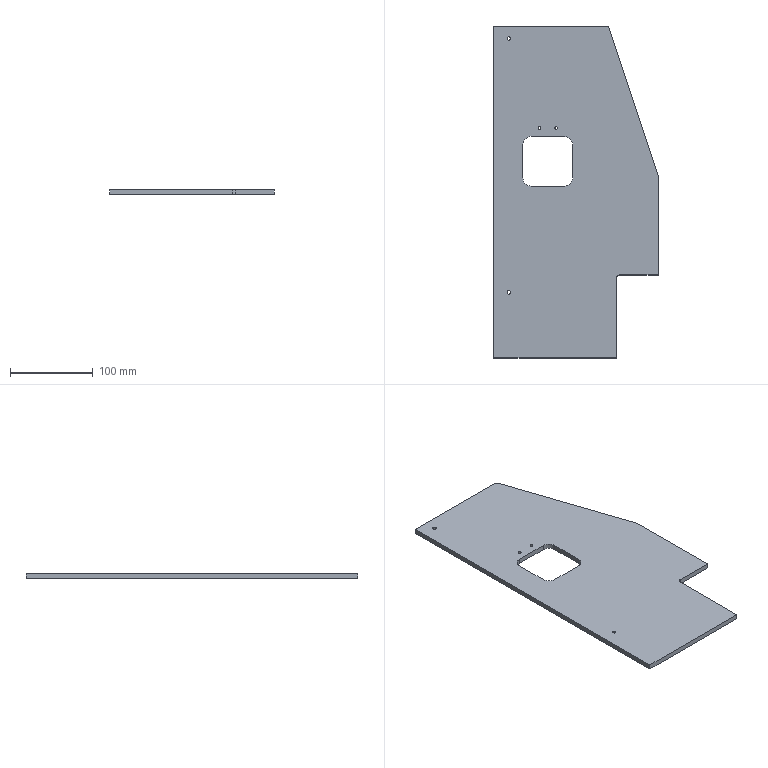Component | SolidWorks | THK-B1006RightFrontBaffle-1 | 1 solid | 28 faces | box 198 x 400 x 6 mm | volume 391453 mm3 | cylinder 15 | plane 13 | commonest cylinder face diameters 3.3 x4 4.2 x4 20 x4 8 x2 7 x1 | material Q235A
build123d program:
from build123d import *

# Parameters (mm, degrees)
BOSS_EXTRUDE1_DEPTH = 3
M5_TAPPED_HOLE1_D   = 4.2
FILLET1_R           = 4
M4_TAPPED_HOLE1_D   = 3.3


with BuildPart() as part:
    # Sketch1 → Boss-Extrude1 (new, symmetric)
    with BuildSketch(Plane(origin=(0, 0, 0), x_dir=(-1, 0, 0), z_dir=(0, 0, -1))):
        with BuildLine():
            Line((-99, 200), (39, 200))
            Line((39, 200), (99, 20))
            Line((99, 20), (99, -100))
            Line((99, -100), (52.5, -100))
            ThreePointArc((52.5, -100), (50.025, -101.025), (49, -103.5))
            Line((49, -103.5), (49, -200))
            Line((49, -200), (-99, -200))
            Line((-99, -200), (-99, 200))
        make_face()
        with BuildLine():
            Line((-14, 67), (-54, 67))
            ThreePointArc((-54, 67), (-61.071, 64.071), (-64, 57))
            Line((-64, 57), (-64, 17))
            ThreePointArc((-64, 17), (-61.071, 9.929), (-54, 7))
            Line((-54, 7), (-14, 7))
            ThreePointArc((-14, 7), (-6.929, 9.929), (-4, 17))
            Line((-4, 17), (-4, 57))
            ThreePointArc((-4, 57), (-6.929, 64.071), (-14, 67))
        make_face(mode=Mode.SUBTRACT)
    extrude(amount=BOSS_EXTRUDE1_DEPTH, both=True)

    # M5 Tapped Hole1 (through all)
    with Locations(Plane(origin=(0, 0, -3), x_dir=(-1, 0, 0), z_dir=(0, 0, -1))):
        with Locations((-81, 185), (-81, -121)):
            Hole(M5_TAPPED_HOLE1_D / 2)

    # Fillet1
    fillet1_edges = [part.edges().sort_by_distance(p)[0] for p in [
        (-39, 200, 0),
        (-99, 20, 0),
    ]]
    fillet(fillet1_edges, radius=FILLET1_R)

    # M4 Tapped Hole1 (through all)
    with Locations(Plane.XY.offset(3)):
        with Locations((24, 77), (44, 77)):
            Hole(M4_TAPPED_HOLE1_D / 2)


solid = part.part

# Placed as in the assembly
solid = solid.moved(Location((221, 0, -258), (-180, 0, 180)))
STEP:
#1=COLOUR_RGB('',0.7922,0.8196,0.9333);
#2=FILL_AREA_STYLE_COLOUR('',#1);
#3=FILL_AREA_STYLE('',(#2));
#4=SURFACE_STYLE_FILL_AREA(#3);
#5=SURFACE_SIDE_STYLE('',(#4));
#6=SURFACE_STYLE_USAGE(.BOTH.,#5);
#7=PRESENTATION_STYLE_ASSIGNMENT((#6));
#8=CARTESIAN_POINT('',(7.821,3.031,-10.039));
#9=VERTEX_POINT('',#8);
#10=CARTESIAN_POINT('',(7.691,3.031,-10.039));
#11=VERTEX_POINT('',#10);
#12=CARTESIAN_POINT('',(7.756,3.031,-10.039));
#13=DIRECTION('',(0.,-0.,-1.));
#14=DIRECTION('',(-1.,0.,0.));
#15=AXIS2_PLACEMENT_3D('',#12,#13,#14);
#16=CIRCLE('',#15,0.06496);
#17=EDGE_CURVE('',#9,#11,#16,.T.);
#18=ORIENTED_EDGE('',*,*,#17,.F.);
#19=CARTESIAN_POINT('',(7.821,3.031,-10.276));
#20=VERTEX_POINT('',#19);
#21=CARTESIAN_POINT('',(7.821,3.031,-10.276));
#22=DIRECTION('',(0.,-0.,-1.));
#23=VECTOR('',#22,39.37);
#24=LINE('',#21,#23);
#25=EDGE_CURVE('',#9,#20,#24,.T.);
#26=ORIENTED_EDGE('',*,*,#25,.T.);
#27=CARTESIAN_POINT('',(7.691,3.031,-10.276));
#28=VERTEX_POINT('',#27);
#29=CARTESIAN_POINT('',(7.756,3.031,-10.276));
#30=DIRECTION('',(0.,-0.,-1.));
#31=DIRECTION('',(-1.,0.,0.));
#32=AXIS2_PLACEMENT_3D('',#29,#30,#31);
#33=CIRCLE('',#32,0.06496);
#34=EDGE_CURVE('',#20,#28,#33,.T.);
#35=ORIENTED_EDGE('',*,*,#34,.T.);
#36=CARTESIAN_POINT('',(7.691,3.031,-10.276));
#37=DIRECTION('',(0.,-0.,-1.));
#38=VECTOR('',#37,39.37);
#39=LINE('',#36,#38);
#40=EDGE_CURVE('',#11,#28,#39,.T.);
#41=ORIENTED_EDGE('',*,*,#40,.F.);
#42=EDGE_LOOP('',(#18,#26,#35,#41));
#43=FACE_OUTER_BOUND('',#42,.T.);
#44=CARTESIAN_POINT('',(7.756,3.031,-10.276));
#45=DIRECTION('',(0.,-0.,-1.));
#46=DIRECTION('',(-1.,0.,0.));
#47=AXIS2_PLACEMENT_3D('',#44,#45,#46);
#48=CYLINDRICAL_SURFACE('',#47,0.06496);
#49=ADVANCED_FACE('',(#43),#48,.F.);
#50=CARTESIAN_POINT('',(7.033,3.031,-10.039));
#51=VERTEX_POINT('',#50);
#52=CARTESIAN_POINT('',(6.904,3.031,-10.039));
#53=VERTEX_POINT('',#52);
#54=CARTESIAN_POINT('',(6.969,3.031,-10.039));
#55=DIRECTION('',(0.,-0.,-1.));
#56=DIRECTION('',(-1.,0.,0.));
#57=AXIS2_PLACEMENT_3D('',#54,#55,#56);
#58=CIRCLE('',#57,0.06496);
#59=EDGE_CURVE('',#51,#53,#58,.T.);
#60=ORIENTED_EDGE('',*,*,#59,.F.);
#61=CARTESIAN_POINT('',(7.033,3.031,-10.276));
#62=VERTEX_POINT('',#61);
#63=CARTESIAN_POINT('',(7.033,3.031,-10.276));
#64=DIRECTION('',(0.,-0.,-1.));
#65=VECTOR('',#64,39.37);
#66=LINE('',#63,#65);
#67=EDGE_CURVE('',#51,#62,#66,.T.);
#68=ORIENTED_EDGE('',*,*,#67,.T.);
#69=CARTESIAN_POINT('',(6.904,3.031,-10.276));
#70=VERTEX_POINT('',#69);
#71=CARTESIAN_POINT('',(6.969,3.031,-10.276));
#72=DIRECTION('',(0.,-0.,-1.));
#73=DIRECTION('',(-1.,0.,0.));
#74=AXIS2_PLACEMENT_3D('',#71,#72,#73);
#75=CIRCLE('',#74,0.06496);
#76=EDGE_CURVE('',#62,#70,#75,.T.);
#77=ORIENTED_EDGE('',*,*,#76,.T.);
#78=CARTESIAN_POINT('',(6.904,3.031,-10.276));
#79=DIRECTION('',(0.,-0.,-1.));
#80=VECTOR('',#79,39.37);
#81=LINE('',#78,#80);
#82=EDGE_CURVE('',#53,#70,#81,.T.);
#83=ORIENTED_EDGE('',*,*,#82,.F.);
#84=EDGE_LOOP('',(#60,#68,#77,#83));
#85=FACE_OUTER_BOUND('',#84,.T.);
#86=CARTESIAN_POINT('',(6.969,3.031,-10.276));
#87=DIRECTION('',(0.,-0.,-1.));
#88=DIRECTION('',(-1.,0.,0.));
#89=AXIS2_PLACEMENT_3D('',#86,#87,#88);
#90=CYLINDRICAL_SURFACE('',#89,0.06496);
#91=ADVANCED_FACE('',(#85),#90,.F.);
#92=CARTESIAN_POINT('',(5.429,7.283,-10.276));
#93=VERTEX_POINT('',#92);
#94=CARTESIAN_POINT('',(5.594,7.283,-10.276));
#95=VERTEX_POINT('',#94);
#96=CARTESIAN_POINT('',(5.512,7.283,-10.276));
#97=DIRECTION('',(-0.,0.,1.));
#98=DIRECTION('',(1.,0.,0.));
#99=AXIS2_PLACEMENT_3D('',#96,#97,#98);
#100=CIRCLE('',#99,0.08268);
#101=EDGE_CURVE('',#93,#95,#100,.T.);
#102=ORIENTED_EDGE('',*,*,#101,.F.);
#103=CARTESIAN_POINT('',(5.429,7.283,-10.039));
#104=VERTEX_POINT('',#103);
#105=CARTESIAN_POINT('',(5.429,7.283,-10.039));
#106=DIRECTION('',(-0.,0.,1.));
#107=VECTOR('',#106,39.37);
#108=LINE('',#105,#107);
#109=EDGE_CURVE('',#93,#104,#108,.T.);
#110=ORIENTED_EDGE('',*,*,#109,.T.);
#111=CARTESIAN_POINT('',(5.594,7.283,-10.039));
#112=VERTEX_POINT('',#111);
#113=CARTESIAN_POINT('',(5.512,7.283,-10.039));
#114=DIRECTION('',(-0.,0.,1.));
#115=DIRECTION('',(1.,0.,0.));
#116=AXIS2_PLACEMENT_3D('',#113,#114,#115);
#117=CIRCLE('',#116,0.08268);
#118=EDGE_CURVE('',#104,#112,#117,.T.);
#119=ORIENTED_EDGE('',*,*,#118,.T.);
#120=CARTESIAN_POINT('',(5.594,7.283,-10.039));
#121=DIRECTION('',(-0.,0.,1.));
#122=VECTOR('',#121,39.37);
#123=LINE('',#120,#122);
#124=EDGE_CURVE('',#95,#112,#123,.T.);
#125=ORIENTED_EDGE('',*,*,#124,.F.);
#126=EDGE_LOOP('',(#102,#110,#119,#125));
#127=FACE_OUTER_BOUND('',#126,.T.);
#128=CARTESIAN_POINT('',(5.512,7.283,-10.039));
#129=DIRECTION('',(-0.,0.,1.));
#130=DIRECTION('',(1.,0.,0.));
#131=AXIS2_PLACEMENT_3D('',#128,#129,#130);
#132=CYLINDRICAL_SURFACE('',#131,0.08268);
#133=ADVANCED_FACE('',(#127),#132,.F.);
#134=CARTESIAN_POINT('',(5.429,-4.764,-10.276));
#135=VERTEX_POINT('',#134);
#136=CARTESIAN_POINT('',(5.594,-4.764,-10.276));
#137=VERTEX_POINT('',#136);
#138=CARTESIAN_POINT('',(5.512,-4.764,-10.276));
#139=DIRECTION('',(-0.,0.,1.));
#140=DIRECTION('',(1.,0.,0.));
#141=AXIS2_PLACEMENT_3D('',#138,#139,#140);
#142=CIRCLE('',#141,0.08268);
#143=EDGE_CURVE('',#135,#137,#142,.T.);
#144=ORIENTED_EDGE('',*,*,#143,.F.);
#145=CARTESIAN_POINT('',(5.429,-4.764,-10.039));
#146=VERTEX_POINT('',#145);
#147=CARTESIAN_POINT('',(5.429,-4.764,-10.039));
#148=DIRECTION('',(-0.,0.,1.));
#149=VECTOR('',#148,39.37);
#150=LINE('',#147,#149);
#151=EDGE_CURVE('',#135,#146,#150,.T.);
#152=ORIENTED_EDGE('',*,*,#151,.T.);
#153=CARTESIAN_POINT('',(5.594,-4.764,-10.039));
#154=VERTEX_POINT('',#153);
#155=CARTESIAN_POINT('',(5.512,-4.764,-10.039));
#156=DIRECTION('',(-0.,0.,1.));
#157=DIRECTION('',(1.,0.,0.));
#158=AXIS2_PLACEMENT_3D('',#155,#156,#157);
#159=CIRCLE('',#158,0.08268);
#160=EDGE_CURVE('',#146,#154,#159,.T.);
#161=ORIENTED_EDGE('',*,*,#160,.T.);
#162=CARTESIAN_POINT('',(5.594,-4.764,-10.039));
#163=DIRECTION('',(-0.,0.,1.));
#164=VECTOR('',#163,39.37);
#165=LINE('',#162,#164);
#166=EDGE_CURVE('',#137,#154,#165,.T.);
#167=ORIENTED_EDGE('',*,*,#166,.F.);
#168=EDGE_LOOP('',(#144,#152,#161,#167));
#169=FACE_OUTER_BOUND('',#168,.T.);
#170=CARTESIAN_POINT('',(5.512,-4.764,-10.039));
#171=DIRECTION('',(-0.,0.,1.));
#172=DIRECTION('',(1.,0.,0.));
#173=AXIS2_PLACEMENT_3D('',#170,#171,#172);
#174=CYLINDRICAL_SURFACE('',#173,0.08268);
#175=ADVANCED_FACE('',(#169),#174,.F.);
#176=CARTESIAN_POINT('',(7.756,3.031,-10.039));
#177=DIRECTION('',(0.,-0.,-1.));
#178=DIRECTION('',(-1.,0.,0.));
#179=AXIS2_PLACEMENT_3D('',#176,#177,#178);
#180=CIRCLE('',#179,0.06496);
#181=EDGE_CURVE('',#11,#9,#180,.T.);
#182=ORIENTED_EDGE('',*,*,#181,.T.);
#183=ORIENTED_EDGE('',*,*,#17,.T.);
#184=EDGE_LOOP('',(#182,#183));
#185=FACE_BOUND('',#184,.T.);
#186=CARTESIAN_POINT('',(6.969,3.031,-10.039));
#187=DIRECTION('',(0.,-0.,-1.));
#188=DIRECTION('',(-1.,0.,0.));
#189=AXIS2_PLACEMENT_3D('',#186,#187,#188);
#190=CIRCLE('',#189,0.06496);
#191=EDGE_CURVE('',#53,#51,#190,.T.);
#192=ORIENTED_EDGE('',*,*,#191,.T.);
#193=ORIENTED_EDGE('',*,*,#59,.T.);
#194=EDGE_LOOP('',(#192,#193));
#195=FACE_BOUND('',#194,.T.);
#196=CARTESIAN_POINT('',(5.512,7.283,-10.039));
#197=DIRECTION('',(-0.,0.,1.));
#198=DIRECTION('',(1.,0.,0.));
#199=AXIS2_PLACEMENT_3D('',#196,#197,#198);
#200=CIRCLE('',#199,0.08268);
#201=EDGE_CURVE('',#112,#104,#200,.T.);
#202=ORIENTED_EDGE('',*,*,#201,.F.);
#203=ORIENTED_EDGE('',*,*,#118,.F.);
#204=EDGE_LOOP('',(#202,#203));
#205=FACE_BOUND('',#204,.T.);
#206=CARTESIAN_POINT('',(5.512,-4.764,-10.039));
#207=DIRECTION('',(-0.,0.,1.));
#208=DIRECTION('',(1.,0.,0.));
#209=AXIS2_PLACEMENT_3D('',#206,#207,#208);
#210=CIRCLE('',#209,0.08268);
#211=EDGE_CURVE('',#154,#146,#210,.T.);
#212=ORIENTED_EDGE('',*,*,#211,.F.);
#213=ORIENTED_EDGE('',*,*,#160,.F.);
#214=EDGE_LOOP('',(#212,#213));
#215=FACE_BOUND('',#214,.T.);
#216=CARTESIAN_POINT('',(12.598,-3.937,-10.039));
#217=VERTEX_POINT('',#216);
#218=CARTESIAN_POINT('',(12.598,0.7618,-10.039));
#219=VERTEX_POINT('',#218);
#220=CARTESIAN_POINT('',(12.598,0.7874,-10.039));
#221=DIRECTION('',(-0.,1.,-0.));
#222=VECTOR('',#221,39.37);
#223=LINE('',#220,#222);
#224=EDGE_CURVE('',#217,#219,#223,.T.);
#225=ORIENTED_EDGE('',*,*,#224,.T.);
#226=CARTESIAN_POINT('',(12.59,0.8116,-10.039));
#227=VERTEX_POINT('',#226);
#228=CARTESIAN_POINT('',(12.441,0.7618,-10.039));
#229=DIRECTION('',(-0.,0.,1.));
#230=DIRECTION('',(-1.,0.,0.));
#231=AXIS2_PLACEMENT_3D('',#228,#229,#230);
#232=CIRCLE('',#231,0.1575);
#233=EDGE_CURVE('',#219,#227,#232,.T.);
#234=ORIENTED_EDGE('',*,*,#233,.T.);
#235=CARTESIAN_POINT('',(10.272,7.766,-10.039));
#236=VERTEX_POINT('',#235);
#237=CARTESIAN_POINT('',(10.236,7.874,-10.039));
#238=DIRECTION('',(-0.3162,0.9487,-0.));
#239=VECTOR('',#238,39.37);
#240=LINE('',#237,#239);
#241=EDGE_CURVE('',#227,#236,#240,.T.);
#242=ORIENTED_EDGE('',*,*,#241,.T.);
#243=CARTESIAN_POINT('',(10.123,7.874,-10.039));
#244=VERTEX_POINT('',#243);
#245=CARTESIAN_POINT('',(10.123,7.717,-10.039));
#246=DIRECTION('',(-0.,0.,1.));
#247=DIRECTION('',(-1.,0.,0.));
#248=AXIS2_PLACEMENT_3D('',#245,#246,#247);
#249=CIRCLE('',#248,0.1575);
#250=EDGE_CURVE('',#236,#244,#249,.T.);
#251=ORIENTED_EDGE('',*,*,#250,.T.);
#252=CARTESIAN_POINT('',(4.803,7.874,-10.039));
#253=VERTEX_POINT('',#252);
#254=CARTESIAN_POINT('',(4.803,7.874,-10.039));
#255=DIRECTION('',(-1.,0.,-0.));
#256=VECTOR('',#255,39.37);
#257=LINE('',#254,#256);
#258=EDGE_CURVE('',#244,#253,#257,.T.);
#259=ORIENTED_EDGE('',*,*,#258,.T.);
#260=CARTESIAN_POINT('',(4.803,-7.874,-10.039));
#261=VERTEX_POINT('',#260);
#262=CARTESIAN_POINT('',(4.803,-7.874,-10.039));
#263=DIRECTION('',(0.,-1.,0.));
#264=VECTOR('',#263,39.37);
#265=LINE('',#262,#264);
#266=EDGE_CURVE('',#253,#261,#265,.T.);
#267=ORIENTED_EDGE('',*,*,#266,.T.);
#268=CARTESIAN_POINT('',(10.63,-7.874,-10.039));
#269=VERTEX_POINT('',#268);
#270=CARTESIAN_POINT('',(10.63,-7.874,-10.039));
#271=DIRECTION('',(1.,0.,0.));
#272=VECTOR('',#271,39.37);
#273=LINE('',#270,#272);
#274=EDGE_CURVE('',#261,#269,#273,.T.);
#275=ORIENTED_EDGE('',*,*,#274,.T.);
#276=CARTESIAN_POINT('',(10.63,-4.075,-10.039));
#277=VERTEX_POINT('',#276);
#278=CARTESIAN_POINT('',(10.63,-7.874,-10.039));
#279=DIRECTION('',(-0.,1.,-0.));
#280=VECTOR('',#279,39.37);
#281=LINE('',#278,#280);
#282=EDGE_CURVE('',#269,#277,#281,.T.);
#283=ORIENTED_EDGE('',*,*,#282,.T.);
#284=CARTESIAN_POINT('',(10.768,-3.937,-10.039));
#285=VERTEX_POINT('',#284);
#286=CARTESIAN_POINT('',(10.768,-4.075,-10.039));
#287=DIRECTION('',(0.,-0.,-1.));
#288=DIRECTION('',(-1.,0.,0.));
#289=AXIS2_PLACEMENT_3D('',#286,#287,#288);
#290=CIRCLE('',#289,0.1378);
#291=EDGE_CURVE('',#277,#285,#290,.T.);
#292=ORIENTED_EDGE('',*,*,#291,.T.);
#293=CARTESIAN_POINT('',(10.768,-3.937,-10.039));
#294=DIRECTION('',(1.,0.,0.));
#295=VECTOR('',#294,39.37);
#296=LINE('',#293,#295);
#297=EDGE_CURVE('',#285,#217,#296,.T.);
#298=ORIENTED_EDGE('',*,*,#297,.T.);
#299=EDGE_LOOP('',(#225,#234,#242,#251,#259,#267,#275,#283,#292,#298));
#300=FACE_OUTER_BOUND('',#299,.T.);
#301=CARTESIAN_POINT('',(6.575,2.638,-10.039));
#302=VERTEX_POINT('',#301);
#303=CARTESIAN_POINT('',(6.181,2.244,-10.039));
#304=VERTEX_POINT('',#303);
#305=CARTESIAN_POINT('',(6.575,2.244,-10.039));
#306=DIRECTION('',(-0.,0.,1.));
#307=DIRECTION('',(1.,0.,0.));
#308=AXIS2_PLACEMENT_3D('',#305,#306,#307);
#309=CIRCLE('',#308,0.3937);
#310=EDGE_CURVE('',#302,#304,#309,.T.);
#311=ORIENTED_EDGE('',*,*,#310,.F.);
#312=CARTESIAN_POINT('',(8.15,2.638,-10.039));
#313=VERTEX_POINT('',#312);
#314=CARTESIAN_POINT('',(8.15,2.638,-10.039));
#315=DIRECTION('',(-1.,-0.,-0.));
#316=VECTOR('',#315,39.37);
#317=LINE('',#314,#316);
#318=EDGE_CURVE('',#313,#302,#317,.T.);
#319=ORIENTED_EDGE('',*,*,#318,.F.);
#320=CARTESIAN_POINT('',(8.543,2.244,-10.039));
#321=VERTEX_POINT('',#320);
#322=CARTESIAN_POINT('',(8.15,2.244,-10.039));
#323=DIRECTION('',(-0.,0.,1.));
#324=DIRECTION('',(1.,0.,0.));
#325=AXIS2_PLACEMENT_3D('',#322,#323,#324);
#326=CIRCLE('',#325,0.3937);
#327=EDGE_CURVE('',#321,#313,#326,.T.);
#328=ORIENTED_EDGE('',*,*,#327,.F.);
#329=CARTESIAN_POINT('',(8.543,0.6693,-10.039));
#330=VERTEX_POINT('',#329);
#331=CARTESIAN_POINT('',(8.543,2.244,-10.039));
#332=DIRECTION('',(-0.,1.,-0.));
#333=VECTOR('',#332,39.37);
#334=LINE('',#331,#333);
#335=EDGE_CURVE('',#330,#321,#334,.T.);
#336=ORIENTED_EDGE('',*,*,#335,.F.);
#337=CARTESIAN_POINT('',(8.15,0.2756,-10.039));
#338=VERTEX_POINT('',#337);
#339=CARTESIAN_POINT('',(8.15,0.6693,-10.039));
#340=DIRECTION('',(-0.,0.,1.));
#341=DIRECTION('',(-1.,0.,0.));
#342=AXIS2_PLACEMENT_3D('',#339,#340,#341);
#343=CIRCLE('',#342,0.3937);
#344=EDGE_CURVE('',#338,#330,#343,.T.);
#345=ORIENTED_EDGE('',*,*,#344,.F.);
#346=CARTESIAN_POINT('',(6.575,0.2756,-10.039));
#347=VERTEX_POINT('',#346);
#348=CARTESIAN_POINT('',(8.15,0.2756,-10.039));
#349=DIRECTION('',(1.,0.,0.));
#350=VECTOR('',#349,39.37);
#351=LINE('',#348,#350);
#352=EDGE_CURVE('',#347,#338,#351,.T.);
#353=ORIENTED_EDGE('',*,*,#352,.F.);
#354=CARTESIAN_POINT('',(6.181,0.6693,-10.039));
#355=VERTEX_POINT('',#354);
#356=CARTESIAN_POINT('',(6.575,0.6693,-10.039));
#357=DIRECTION('',(-0.,0.,1.));
#358=DIRECTION('',(1.,0.,0.));
#359=AXIS2_PLACEMENT_3D('',#356,#357,#358);
#360=CIRCLE('',#359,0.3937);
#361=EDGE_CURVE('',#355,#347,#360,.T.);
#362=ORIENTED_EDGE('',*,*,#361,.F.);
#363=CARTESIAN_POINT('',(6.181,2.244,-10.039));
#364=DIRECTION('',(0.,-1.,0.));
#365=VECTOR('',#364,39.37);
#366=LINE('',#363,#365);
#367=EDGE_CURVE('',#304,#355,#366,.T.);
#368=ORIENTED_EDGE('',*,*,#367,.F.);
#369=EDGE_LOOP('',(#311,#319,#328,#336,#345,#353,#362,#368));
#370=FACE_BOUND('',#369,.T.);
#371=CARTESIAN_POINT('',(10.768,-4.075,-10.039));
#372=DIRECTION('',(0.,-0.,-1.));
#373=DIRECTION('',(-1.,-0.,-0.));
#374=AXIS2_PLACEMENT_3D('',#371,#372,#373);
#375=PLANE('',#374);
#376=ADVANCED_FACE('',(#185,#195,#205,#215,#300,#370),#375,.F.);
#377=CARTESIAN_POINT('',(7.756,3.031,-10.276));
#378=DIRECTION('',(0.,-0.,-1.));
#379=DIRECTION('',(-1.,0.,0.));
#380=AXIS2_PLACEMENT_3D('',#377,#378,#379);
#381=CIRCLE('',#380,0.06496);
#382=EDGE_CURVE('',#28,#20,#381,.T.);
#383=ORIENTED_EDGE('',*,*,#382,.F.);
#384=ORIENTED_EDGE('',*,*,#34,.F.);
#385=EDGE_LOOP('',(#383,#384));
#386=FACE_BOUND('',#385,.T.);
#387=CARTESIAN_POINT('',(6.969,3.031,-10.276));
#388=DIRECTION('',(0.,-0.,-1.));
#389=DIRECTION('',(-1.,0.,0.));
#390=AXIS2_PLACEMENT_3D('',#387,#388,#389);
#391=CIRCLE('',#390,0.06496);
#392=EDGE_CURVE('',#70,#62,#391,.T.);
#393=ORIENTED_EDGE('',*,*,#392,.F.);
#394=ORIENTED_EDGE('',*,*,#76,.F.);
#395=EDGE_LOOP('',(#393,#394));
#396=FACE_BOUND('',#395,.T.);
#397=CARTESIAN_POINT('',(5.512,7.283,-10.276));
#398=DIRECTION('',(-0.,0.,1.));
#399=DIRECTION('',(1.,0.,0.));
#400=AXIS2_PLACEMENT_3D('',#397,#398,#399);
#401=CIRCLE('',#400,0.08268);
#402=EDGE_CURVE('',#95,#93,#401,.T.);
#403=ORIENTED_EDGE('',*,*,#402,.T.);
#404=ORIENTED_EDGE('',*,*,#101,.T.);
#405=EDGE_LOOP('',(#403,#404));
#406=FACE_BOUND('',#405,.T.);
#407=CARTESIAN_POINT('',(5.512,-4.764,-10.276));
#408=DIRECTION('',(-0.,0.,1.));
#409=DIRECTION('',(1.,0.,0.));
#410=AXIS2_PLACEMENT_3D('',#407,#408,#409);
#411=CIRCLE('',#410,0.08268);
#412=EDGE_CURVE('',#137,#135,#411,.T.);
#413=ORIENTED_EDGE('',*,*,#412,.T.);
#414=ORIENTED_EDGE('',*,*,#143,.T.);
#415=EDGE_LOOP('',(#413,#414));
#416=FACE_BOUND('',#415,.T.);
#417=CARTESIAN_POINT('',(12.59,0.8116,-10.276));
#418=VERTEX_POINT('',#417);
#419=CARTESIAN_POINT('',(10.272,7.766,-10.276));
#420=VERTEX_POINT('',#419);
#421=CARTESIAN_POINT('',(10.236,7.874,-10.276));
#422=DIRECTION('',(-0.3162,0.9487,-0.));
#423=VECTOR('',#422,39.37);
#424=LINE('',#421,#423);
#425=EDGE_CURVE('',#418,#420,#424,.T.);
#426=ORIENTED_EDGE('',*,*,#425,.F.);
#427=CARTESIAN_POINT('',(12.598,0.7618,-10.276));
#428=VERTEX_POINT('',#427);
#429=CARTESIAN_POINT('',(12.441,0.7618,-10.276));
#430=DIRECTION('',(0.,-0.,-1.));
#431=DIRECTION('',(-1.,0.,0.));
#432=AXIS2_PLACEMENT_3D('',#429,#430,#431);
#433=CIRCLE('',#432,0.1575);
#434=EDGE_CURVE('',#418,#428,#433,.T.);
#435=ORIENTED_EDGE('',*,*,#434,.T.);
#436=CARTESIAN_POINT('',(12.598,-3.937,-10.276));
#437=VERTEX_POINT('',#436);
#438=CARTESIAN_POINT('',(12.598,0.7874,-10.276));
#439=DIRECTION('',(-0.,1.,-0.));
#440=VECTOR('',#439,39.37);
#441=LINE('',#438,#440);
#442=EDGE_CURVE('',#437,#428,#441,.T.);
#443=ORIENTED_EDGE('',*,*,#442,.F.);
#444=CARTESIAN_POINT('',(10.768,-3.937,-10.276));
#445=VERTEX_POINT('',#444);
#446=CARTESIAN_POINT('',(10.768,-3.937,-10.276));
#447=DIRECTION('',(1.,0.,0.));
#448=VECTOR('',#447,39.37);
#449=LINE('',#446,#448);
#450=EDGE_CURVE('',#445,#437,#449,.T.);
#451=ORIENTED_EDGE('',*,*,#450,.F.);
#452=CARTESIAN_POINT('',(10.63,-4.075,-10.276));
#453=VERTEX_POINT('',#452);
#454=CARTESIAN_POINT('',(10.768,-4.075,-10.276));
#455=DIRECTION('',(0.,-0.,-1.));
#456=DIRECTION('',(-1.,0.,0.));
#457=AXIS2_PLACEMENT_3D('',#454,#455,#456);
#458=CIRCLE('',#457,0.1378);
#459=EDGE_CURVE('',#453,#445,#458,.T.);
#460=ORIENTED_EDGE('',*,*,#459,.F.);
#461=CARTESIAN_POINT('',(10.63,-7.874,-10.276));
#462=VERTEX_POINT('',#461);
#463=CARTESIAN_POINT('',(10.63,-7.874,-10.276));
#464=DIRECTION('',(-0.,1.,-0.));
#465=VECTOR('',#464,39.37);
#466=LINE('',#463,#465);
#467=EDGE_CURVE('',#462,#453,#466,.T.);
#468=ORIENTED_EDGE('',*,*,#467,.F.);
#469=CARTESIAN_POINT('',(4.803,-7.874,-10.276));
#470=VERTEX_POINT('',#469);
#471=CARTESIAN_POINT('',(10.63,-7.874,-10.276));
#472=DIRECTION('',(1.,0.,0.));
#473=VECTOR('',#472,39.37);
#474=LINE('',#471,#473);
#475=EDGE_CURVE('',#470,#462,#474,.T.);
#476=ORIENTED_EDGE('',*,*,#475,.F.);
#477=CARTESIAN_POINT('',(4.803,7.874,-10.276));
#478=VERTEX_POINT('',#477);
#479=CARTESIAN_POINT('',(4.803,-7.874,-10.276));
#480=DIRECTION('',(0.,-1.,0.));
#481=VECTOR('',#480,39.37);
#482=LINE('',#479,#481);
#483=EDGE_CURVE('',#478,#470,#482,.T.);
#484=ORIENTED_EDGE('',*,*,#483,.F.);
#485=CARTESIAN_POINT('',(10.123,7.874,-10.276));
#486=VERTEX_POINT('',#485);
#487=CARTESIAN_POINT('',(4.803,7.874,-10.276));
#488=DIRECTION('',(-1.,0.,-0.));
#489=VECTOR('',#488,39.37);
#490=LINE('',#487,#489);
#491=EDGE_CURVE('',#486,#478,#490,.T.);
#492=ORIENTED_EDGE('',*,*,#491,.F.);
#493=CARTESIAN_POINT('',(10.123,7.717,-10.276));
#494=DIRECTION('',(0.,-0.,-1.));
#495=DIRECTION('',(-1.,0.,0.));
#496=AXIS2_PLACEMENT_3D('',#493,#494,#495);
#497=CIRCLE('',#496,0.1575);
#498=EDGE_CURVE('',#486,#420,#497,.T.);
#499=ORIENTED_EDGE('',*,*,#498,.T.);
#500=EDGE_LOOP('',(#426,#435,#443,#451,#460,#468,#476,#484,#492,#499));
#501=FACE_OUTER_BOUND('',#500,.T.);
#502=CARTESIAN_POINT('',(8.15,2.638,-10.276));
#503=VERTEX_POINT('',#502);
#504=CARTESIAN_POINT('',(6.575,2.638,-10.276));
#505=VERTEX_POINT('',#504);
#506=CARTESIAN_POINT('',(8.15,2.638,-10.276));
#507=DIRECTION('',(-1.,-0.,-0.));
#508=VECTOR('',#507,39.37);
#509=LINE('',#506,#508);
#510=EDGE_CURVE('',#503,#505,#509,.T.);
#511=ORIENTED_EDGE('',*,*,#510,.T.);
#512=CARTESIAN_POINT('',(6.181,2.244,-10.276));
#513=VERTEX_POINT('',#512);
#514=CARTESIAN_POINT('',(6.575,2.244,-10.276));
#515=DIRECTION('',(-0.,0.,1.));
#516=DIRECTION('',(1.,0.,0.));
#517=AXIS2_PLACEMENT_3D('',#514,#515,#516);
#518=CIRCLE('',#517,0.3937);
#519=EDGE_CURVE('',#505,#513,#518,.T.);
#520=ORIENTED_EDGE('',*,*,#519,.T.);
#521=CARTESIAN_POINT('',(6.181,0.6693,-10.276));
#522=VERTEX_POINT('',#521);
#523=CARTESIAN_POINT('',(6.181,2.244,-10.276));
#524=DIRECTION('',(0.,-1.,0.));
#525=VECTOR('',#524,39.37);
#526=LINE('',#523,#525);
#527=EDGE_CURVE('',#513,#522,#526,.T.);
#528=ORIENTED_EDGE('',*,*,#527,.T.);
#529=CARTESIAN_POINT('',(6.575,0.2756,-10.276));
#530=VERTEX_POINT('',#529);
#531=CARTESIAN_POINT('',(6.575,0.6693,-10.276));
#532=DIRECTION('',(-0.,0.,1.));
#533=DIRECTION('',(1.,0.,0.));
#534=AXIS2_PLACEMENT_3D('',#531,#532,#533);
#535=CIRCLE('',#534,0.3937);
#536=EDGE_CURVE('',#522,#530,#535,.T.);
#537=ORIENTED_EDGE('',*,*,#536,.T.);
#538=CARTESIAN_POINT('',(8.15,0.2756,-10.276));
#539=VERTEX_POINT('',#538);
#540=CARTESIAN_POINT('',(8.15,0.2756,-10.276));
#541=DIRECTION('',(1.,0.,0.));
#542=VECTOR('',#541,39.37);
#543=LINE('',#540,#542);
#544=EDGE_CURVE('',#530,#539,#543,.T.);
#545=ORIENTED_EDGE('',*,*,#544,.T.);
#546=CARTESIAN_POINT('',(8.543,0.6693,-10.276));
#547=VERTEX_POINT('',#546);
#548=CARTESIAN_POINT('',(8.15,0.6693,-10.276));
#549=DIRECTION('',(-0.,0.,1.));
#550=DIRECTION('',(-1.,0.,0.));
#551=AXIS2_PLACEMENT_3D('',#548,#549,#550);
#552=CIRCLE('',#551,0.3937);
#553=EDGE_CURVE('',#539,#547,#552,.T.);
#554=ORIENTED_EDGE('',*,*,#553,.T.);
#555=CARTESIAN_POINT('',(8.543,2.244,-10.276));
#556=VERTEX_POINT('',#555);
#557=CARTESIAN_POINT('',(8.543,2.244,-10.276));
#558=DIRECTION('',(-0.,1.,-0.));
#559=VECTOR('',#558,39.37);
#560=LINE('',#557,#559);
#561=EDGE_CURVE('',#547,#556,#560,.T.);
#562=ORIENTED_EDGE('',*,*,#561,.T.);
#563=CARTESIAN_POINT('',(8.15,2.244,-10.276));
#564=DIRECTION('',(-0.,0.,1.));
#565=DIRECTION('',(1.,0.,0.));
#566=AXIS2_PLACEMENT_3D('',#563,#564,#565);
#567=CIRCLE('',#566,0.3937);
#568=EDGE_CURVE('',#556,#503,#567,.T.);
#569=ORIENTED_EDGE('',*,*,#568,.T.);
#570=EDGE_LOOP('',(#511,#520,#528,#537,#545,#554,#562,#569));
#571=FACE_BOUND('',#570,.T.);
#572=CARTESIAN_POINT('',(10.768,-4.075,-10.276));
#573=DIRECTION('',(0.,-0.,-1.));
#574=DIRECTION('',(-1.,-0.,-0.));
#575=AXIS2_PLACEMENT_3D('',#572,#573,#574);
#576=PLANE('',#575);
#577=ADVANCED_FACE('',(#386,#396,#406,#416,#501,#571),#576,.T.);
#578=ORIENTED_EDGE('',*,*,#442,.T.);
#579=CARTESIAN_POINT('',(12.598,0.7618,-10.039));
#580=DIRECTION('',(-0.,0.,1.));
#581=VECTOR('',#580,39.37);
#582=LINE('',#579,#581);
#583=EDGE_CURVE('',#428,#219,#582,.T.);
#584=ORIENTED_EDGE('',*,*,#583,.T.);
#585=ORIENTED_EDGE('',*,*,#224,.F.);
#586=CARTESIAN_POINT('',(12.598,-3.937,-10.039));
#587=DIRECTION('',(0.,-0.,-1.));
#588=VECTOR('',#587,39.37);
#589=LINE('',#586,#588);
#590=EDGE_CURVE('',#217,#437,#589,.T.);
#591=ORIENTED_EDGE('',*,*,#590,.T.);
#592=EDGE_LOOP('',(#578,#584,#585,#591));
#593=FACE_OUTER_BOUND('',#592,.T.);
#594=CARTESIAN_POINT('',(12.598,0.7874,-10.039));
#595=DIRECTION('',(-1.,-0.,-0.));
#596=DIRECTION('',(-0.,1.,-0.));
#597=AXIS2_PLACEMENT_3D('',#594,#595,#596);
#598=PLANE('',#597);
#599=ADVANCED_FACE('',(#593),#598,.F.);
#600=ORIENTED_EDGE('',*,*,#241,.F.);
#601=CARTESIAN_POINT('',(12.59,0.8116,-10.039));
#602=DIRECTION('',(0.,-0.,-1.));
#603=VECTOR('',#602,39.37);
#604=LINE('',#601,#603);
#605=EDGE_CURVE('',#227,#418,#604,.T.);
#606=ORIENTED_EDGE('',*,*,#605,.T.);
#607=ORIENTED_EDGE('',*,*,#425,.T.);
#608=CARTESIAN_POINT('',(10.272,7.766,-10.039));
#609=DIRECTION('',(-0.,0.,1.));
#610=VECTOR('',#609,39.37);
#611=LINE('',#608,#610);
#612=EDGE_CURVE('',#420,#236,#611,.T.);
#613=ORIENTED_EDGE('',*,*,#612,.T.);
#614=EDGE_LOOP('',(#600,#606,#607,#613));
#615=FACE_OUTER_BOUND('',#614,.T.);
#616=CARTESIAN_POINT('',(10.236,7.874,-10.039));
#617=DIRECTION('',(-0.9487,-0.3162,-0.));
#618=DIRECTION('',(-0.3162,0.9487,-0.));
#619=AXIS2_PLACEMENT_3D('',#616,#617,#618);
#620=PLANE('',#619);
#621=ADVANCED_FACE('',(#615),#620,.F.);
#622=ORIENTED_EDGE('',*,*,#258,.F.);
#623=CARTESIAN_POINT('',(10.123,7.874,-10.039));
#624=DIRECTION('',(0.,-0.,-1.));
#625=VECTOR('',#624,39.37);
#626=LINE('',#623,#625);
#627=EDGE_CURVE('',#244,#486,#626,.T.);
#628=ORIENTED_EDGE('',*,*,#627,.T.);
#629=ORIENTED_EDGE('',*,*,#491,.T.);
#630=CARTESIAN_POINT('',(4.803,7.874,-10.039));
#631=DIRECTION('',(0.,-0.,-1.));
#632=VECTOR('',#631,39.37);
#633=LINE('',#630,#632);
#634=EDGE_CURVE('',#253,#478,#633,.T.);
#635=ORIENTED_EDGE('',*,*,#634,.F.);
#636=EDGE_LOOP('',(#622,#628,#629,#635));
#637=FACE_OUTER_BOUND('',#636,.T.);
#638=CARTESIAN_POINT('',(4.803,7.874,-10.039));
#639=DIRECTION('',(-0.,-1.,0.));
#640=DIRECTION('',(-1.,0.,-0.));
#641=AXIS2_PLACEMENT_3D('',#638,#639,#640);
#642=PLANE('',#641);
#643=ADVANCED_FACE('',(#637),#642,.F.);
#644=ORIENTED_EDGE('',*,*,#483,.T.);
#645=CARTESIAN_POINT('',(4.803,-7.874,-10.039));
#646=DIRECTION('',(0.,-0.,-1.));
#647=VECTOR('',#646,39.37);
#648=LINE('',#645,#647);
#649=EDGE_CURVE('',#261,#470,#648,.T.);
#650=ORIENTED_EDGE('',*,*,#649,.F.);
#651=ORIENTED_EDGE('',*,*,#266,.F.);
#652=ORIENTED_EDGE('',*,*,#634,.T.);
#653=EDGE_LOOP('',(#644,#650,#651,#652));
#654=FACE_OUTER_BOUND('',#653,.T.);
#655=CARTESIAN_POINT('',(4.803,-7.874,-10.039));
#656=DIRECTION('',(1.,0.,0.));
#657=DIRECTION('',(0.,-0.,-1.));
#658=AXIS2_PLACEMENT_3D('',#655,#656,#657);
#659=PLANE('',#658);
#660=ADVANCED_FACE('',(#654),#659,.F.);
#661=ORIENTED_EDGE('',*,*,#475,.T.);
#662=CARTESIAN_POINT('',(10.63,-7.874,-10.039));
#663=DIRECTION('',(0.,-0.,-1.));
#664=VECTOR('',#663,39.37);
#665=LINE('',#662,#664);
#666=EDGE_CURVE('',#269,#462,#665,.T.);
#667=ORIENTED_EDGE('',*,*,#666,.F.);
#668=ORIENTED_EDGE('',*,*,#274,.F.);
#669=ORIENTED_EDGE('',*,*,#649,.T.);
#670=EDGE_LOOP('',(#661,#667,#668,#669));
#671=FACE_OUTER_BOUND('',#670,.T.);
#672=CARTESIAN_POINT('',(10.63,-7.874,-10.039));
#673=DIRECTION('',(-0.,1.,-0.));
#674=DIRECTION('',(1.,0.,0.));
#675=AXIS2_PLACEMENT_3D('',#672,#673,#674);
#676=PLANE('',#675);
#677=ADVANCED_FACE('',(#671),#676,.F.);
#678=ORIENTED_EDGE('',*,*,#467,.T.);
#679=CARTESIAN_POINT('',(10.63,-4.075,-10.039));
#680=DIRECTION('',(0.,-0.,-1.));
#681=VECTOR('',#680,39.37);
#682=LINE('',#679,#681);
#683=EDGE_CURVE('',#277,#453,#682,.T.);
#684=ORIENTED_EDGE('',*,*,#683,.F.);
#685=ORIENTED_EDGE('',*,*,#282,.F.);
#686=ORIENTED_EDGE('',*,*,#666,.T.);
#687=EDGE_LOOP('',(#678,#684,#685,#686));
#688=FACE_OUTER_BOUND('',#687,.T.);
#689=CARTESIAN_POINT('',(10.63,-7.874,-10.039));
#690=DIRECTION('',(-1.,-0.,-0.));
#691=DIRECTION('',(-0.,0.,1.));
#692=AXIS2_PLACEMENT_3D('',#689,#690,#691);
#693=PLANE('',#692);
#694=ADVANCED_FACE('',(#688),#693,.F.);
#695=ORIENTED_EDGE('',*,*,#459,.T.);
#696=CARTESIAN_POINT('',(10.768,-3.937,-10.039));
#697=DIRECTION('',(0.,-0.,-1.));
#698=VECTOR('',#697,39.37);
#699=LINE('',#696,#698);
#700=EDGE_CURVE('',#285,#445,#699,.T.);
#701=ORIENTED_EDGE('',*,*,#700,.F.);
#702=ORIENTED_EDGE('',*,*,#291,.F.);
#703=ORIENTED_EDGE('',*,*,#683,.T.);
#704=EDGE_LOOP('',(#695,#701,#702,#703));
#705=FACE_OUTER_BOUND('',#704,.T.);
#706=CARTESIAN_POINT('',(10.768,-4.075,-10.039));
#707=DIRECTION('',(0.,-0.,-1.));
#708=DIRECTION('',(-1.,0.,0.));
#709=AXIS2_PLACEMENT_3D('',#706,#707,#708);
#710=CYLINDRICAL_SURFACE('',#709,0.1378);
#711=ADVANCED_FACE('',(#705),#710,.F.);
#712=ORIENTED_EDGE('',*,*,#450,.T.);
#713=ORIENTED_EDGE('',*,*,#590,.F.);
#714=ORIENTED_EDGE('',*,*,#297,.F.);
#715=ORIENTED_EDGE('',*,*,#700,.T.);
#716=EDGE_LOOP('',(#712,#713,#714,#715));
#717=FACE_OUTER_BOUND('',#716,.T.);
#718=CARTESIAN_POINT('',(10.768,-3.937,-10.039));
#719=DIRECTION('',(-0.,1.,-0.));
#720=DIRECTION('',(0.,-0.,-1.));
#721=AXIS2_PLACEMENT_3D('',#718,#719,#720);
#722=PLANE('',#721);
#723=ADVANCED_FACE('',(#717),#722,.F.);
#724=ORIENTED_EDGE('',*,*,#519,.F.);
#725=CARTESIAN_POINT('',(6.575,2.638,-10.039));
#726=DIRECTION('',(0.,-0.,-1.));
#727=VECTOR('',#726,39.37);
#728=LINE('',#725,#727);
#729=EDGE_CURVE('',#302,#505,#728,.T.);
#730=ORIENTED_EDGE('',*,*,#729,.F.);
#731=ORIENTED_EDGE('',*,*,#310,.T.);
#732=CARTESIAN_POINT('',(6.181,2.244,-10.039));
#733=DIRECTION('',(0.,-0.,-1.));
#734=VECTOR('',#733,39.37);
#735=LINE('',#732,#734);
#736=EDGE_CURVE('',#304,#513,#735,.T.);
#737=ORIENTED_EDGE('',*,*,#736,.T.);
#738=EDGE_LOOP('',(#724,#730,#731,#737));
#739=FACE_OUTER_BOUND('',#738,.T.);
#740=CARTESIAN_POINT('',(6.575,2.244,-10.039));
#741=DIRECTION('',(0.,-0.,-1.));
#742=DIRECTION('',(-1.,0.,0.));
#743=AXIS2_PLACEMENT_3D('',#740,#741,#742);
#744=CYLINDRICAL_SURFACE('',#743,0.3937);
#745=ADVANCED_FACE('',(#739),#744,.F.);
#746=ORIENTED_EDGE('',*,*,#527,.F.);
#747=ORIENTED_EDGE('',*,*,#736,.F.);
#748=ORIENTED_EDGE('',*,*,#367,.T.);
#749=CARTESIAN_POINT('',(6.181,0.6693,-10.039));
#750=DIRECTION('',(0.,-0.,-1.));
#751=VECTOR('',#750,39.37);
#752=LINE('',#749,#751);
#753=EDGE_CURVE('',#355,#522,#752,.T.);
#754=ORIENTED_EDGE('',*,*,#753,.T.);
#755=EDGE_LOOP('',(#746,#747,#748,#754));
#756=FACE_OUTER_BOUND('',#755,.T.);
#757=CARTESIAN_POINT('',(6.181,2.244,-10.039));
#758=DIRECTION('',(1.,0.,0.));
#759=DIRECTION('',(0.,-1.,0.));
#760=AXIS2_PLACEMENT_3D('',#757,#758,#759);
#761=PLANE('',#760);
#762=ADVANCED_FACE('',(#756),#761,.T.);
#763=ORIENTED_EDGE('',*,*,#536,.F.);
#764=ORIENTED_EDGE('',*,*,#753,.F.);
#765=ORIENTED_EDGE('',*,*,#361,.T.);
#766=CARTESIAN_POINT('',(6.575,0.2756,-10.039));
#767=DIRECTION('',(0.,-0.,-1.));
#768=VECTOR('',#767,39.37);
#769=LINE('',#766,#768);
#770=EDGE_CURVE('',#347,#530,#769,.T.);
#771=ORIENTED_EDGE('',*,*,#770,.T.);
#772=EDGE_LOOP('',(#763,#764,#765,#771));
#773=FACE_OUTER_BOUND('',#772,.T.);
#774=CARTESIAN_POINT('',(6.575,0.6693,-10.039));
#775=DIRECTION('',(0.,-0.,-1.));
#776=DIRECTION('',(-1.,0.,0.));
#777=AXIS2_PLACEMENT_3D('',#774,#775,#776);
#778=CYLINDRICAL_SURFACE('',#777,0.3937);
#779=ADVANCED_FACE('',(#773),#778,.F.);
#780=ORIENTED_EDGE('',*,*,#544,.F.);
#781=ORIENTED_EDGE('',*,*,#770,.F.);
#782=ORIENTED_EDGE('',*,*,#352,.T.);
#783=CARTESIAN_POINT('',(8.15,0.2756,-10.039));
#784=DIRECTION('',(0.,-0.,-1.));
#785=VECTOR('',#784,39.37);
#786=LINE('',#783,#785);
#787=EDGE_CURVE('',#338,#539,#786,.T.);
#788=ORIENTED_EDGE('',*,*,#787,.T.);
#789=EDGE_LOOP('',(#780,#781,#782,#788));
#790=FACE_OUTER_BOUND('',#789,.T.);
#791=CARTESIAN_POINT('',(8.15,0.2756,-10.039));
#792=DIRECTION('',(-0.,1.,-0.));
#793=DIRECTION('',(1.,0.,0.));
#794=AXIS2_PLACEMENT_3D('',#791,#792,#793);
#795=PLANE('',#794);
#796=ADVANCED_FACE('',(#790),#795,.T.);
#797=ORIENTED_EDGE('',*,*,#553,.F.);
#798=ORIENTED_EDGE('',*,*,#787,.F.);
#799=ORIENTED_EDGE('',*,*,#344,.T.);
#800=CARTESIAN_POINT('',(8.543,0.6693,-10.039));
#801=DIRECTION('',(0.,-0.,-1.));
#802=VECTOR('',#801,39.37);
#803=LINE('',#800,#802);
#804=EDGE_CURVE('',#330,#547,#803,.T.);
#805=ORIENTED_EDGE('',*,*,#804,.T.);
#806=EDGE_LOOP('',(#797,#798,#799,#805));
#807=FACE_OUTER_BOUND('',#806,.T.);
#808=CARTESIAN_POINT('',(8.15,0.6693,-10.039));
#809=DIRECTION('',(0.,-0.,-1.));
#810=DIRECTION('',(-1.,0.,0.));
#811=AXIS2_PLACEMENT_3D('',#808,#809,#810);
#812=CYLINDRICAL_SURFACE('',#811,0.3937);
#813=ADVANCED_FACE('',(#807),#812,.F.);
#814=ORIENTED_EDGE('',*,*,#561,.F.);
#815=ORIENTED_EDGE('',*,*,#804,.F.);
#816=ORIENTED_EDGE('',*,*,#335,.T.);
#817=CARTESIAN_POINT('',(8.543,2.244,-10.039));
#818=DIRECTION('',(0.,-0.,-1.));
#819=VECTOR('',#818,39.37);
#820=LINE('',#817,#819);
#821=EDGE_CURVE('',#321,#556,#820,.T.);
#822=ORIENTED_EDGE('',*,*,#821,.T.);
#823=EDGE_LOOP('',(#814,#815,#816,#822));
#824=FACE_OUTER_BOUND('',#823,.T.);
#825=CARTESIAN_POINT('',(8.543,2.244,-10.039));
#826=DIRECTION('',(-1.,-0.,-0.));
#827=DIRECTION('',(-0.,1.,-0.));
#828=AXIS2_PLACEMENT_3D('',#825,#826,#827);
#829=PLANE('',#828);
#830=ADVANCED_FACE('',(#824),#829,.T.);
#831=ORIENTED_EDGE('',*,*,#568,.F.);
#832=ORIENTED_EDGE('',*,*,#821,.F.);
#833=ORIENTED_EDGE('',*,*,#327,.T.);
#834=CARTESIAN_POINT('',(8.15,2.638,-10.039));
#835=DIRECTION('',(0.,-0.,-1.));
#836=VECTOR('',#835,39.37);
#837=LINE('',#834,#836);
#838=EDGE_CURVE('',#313,#503,#837,.T.);
#839=ORIENTED_EDGE('',*,*,#838,.T.);
#840=EDGE_LOOP('',(#831,#832,#833,#839));
#841=FACE_OUTER_BOUND('',#840,.T.);
#842=CARTESIAN_POINT('',(8.15,2.244,-10.039));
#843=DIRECTION('',(0.,-0.,-1.));
#844=DIRECTION('',(-1.,0.,0.));
#845=AXIS2_PLACEMENT_3D('',#842,#843,#844);
#846=CYLINDRICAL_SURFACE('',#845,0.3937);
#847=ADVANCED_FACE('',(#841),#846,.F.);
#848=ORIENTED_EDGE('',*,*,#510,.F.);
#849=ORIENTED_EDGE('',*,*,#838,.F.);
#850=ORIENTED_EDGE('',*,*,#318,.T.);
#851=ORIENTED_EDGE('',*,*,#729,.T.);
#852=EDGE_LOOP('',(#848,#849,#850,#851));
#853=FACE_OUTER_BOUND('',#852,.T.);
#854=CARTESIAN_POINT('',(8.15,2.638,-10.039));
#855=DIRECTION('',(0.,-1.,0.));
#856=DIRECTION('',(-1.,-0.,-0.));
#857=AXIS2_PLACEMENT_3D('',#854,#855,#856);
#858=PLANE('',#857);
#859=ADVANCED_FACE('',(#853),#858,.T.);
#860=ORIENTED_EDGE('',*,*,#151,.F.);
#861=ORIENTED_EDGE('',*,*,#412,.F.);
#862=ORIENTED_EDGE('',*,*,#166,.T.);
#863=ORIENTED_EDGE('',*,*,#211,.T.);
#864=EDGE_LOOP('',(#860,#861,#862,#863));
#865=FACE_OUTER_BOUND('',#864,.T.);
#866=CARTESIAN_POINT('',(5.512,-4.764,-10.039));
#867=DIRECTION('',(-0.,0.,1.));
#868=DIRECTION('',(1.,0.,0.));
#869=AXIS2_PLACEMENT_3D('',#866,#867,#868);
#870=CYLINDRICAL_SURFACE('',#869,0.08268);
#871=ADVANCED_FACE('',(#865),#870,.F.);
#872=ORIENTED_EDGE('',*,*,#109,.F.);
#873=ORIENTED_EDGE('',*,*,#402,.F.);
#874=ORIENTED_EDGE('',*,*,#124,.T.);
#875=ORIENTED_EDGE('',*,*,#201,.T.);
#876=EDGE_LOOP('',(#872,#873,#874,#875));
#877=FACE_OUTER_BOUND('',#876,.T.);
#878=CARTESIAN_POINT('',(5.512,7.283,-10.039));
#879=DIRECTION('',(-0.,0.,1.));
#880=DIRECTION('',(1.,0.,0.));
#881=AXIS2_PLACEMENT_3D('',#878,#879,#880);
#882=CYLINDRICAL_SURFACE('',#881,0.08268);
#883=ADVANCED_FACE('',(#877),#882,.F.);
#884=ORIENTED_EDGE('',*,*,#233,.F.);
#885=ORIENTED_EDGE('',*,*,#583,.F.);
#886=ORIENTED_EDGE('',*,*,#434,.F.);
#887=ORIENTED_EDGE('',*,*,#605,.F.);
#888=EDGE_LOOP('',(#884,#885,#886,#887));
#889=FACE_OUTER_BOUND('',#888,.T.);
#890=CARTESIAN_POINT('',(12.441,0.7618,-10.039));
#891=DIRECTION('',(0.,-0.,-1.));
#892=DIRECTION('',(-1.,0.,0.));
#893=AXIS2_PLACEMENT_3D('',#890,#891,#892);
#894=CYLINDRICAL_SURFACE('',#893,0.1575);
#895=ADVANCED_FACE('',(#889),#894,.T.);
#896=ORIENTED_EDGE('',*,*,#250,.F.);
#897=ORIENTED_EDGE('',*,*,#612,.F.);
#898=ORIENTED_EDGE('',*,*,#498,.F.);
#899=ORIENTED_EDGE('',*,*,#627,.F.);
#900=EDGE_LOOP('',(#896,#897,#898,#899));
#901=FACE_OUTER_BOUND('',#900,.T.);
#902=CARTESIAN_POINT('',(10.123,7.717,-10.039));
#903=DIRECTION('',(0.,-0.,-1.));
#904=DIRECTION('',(-1.,0.,0.));
#905=AXIS2_PLACEMENT_3D('',#902,#903,#904);
#906=CYLINDRICAL_SURFACE('',#905,0.1575);
#907=ADVANCED_FACE('',(#901),#906,.T.);
#908=ORIENTED_EDGE('',*,*,#67,.F.);
#909=ORIENTED_EDGE('',*,*,#191,.F.);
#910=ORIENTED_EDGE('',*,*,#82,.T.);
#911=ORIENTED_EDGE('',*,*,#392,.T.);
#912=EDGE_LOOP('',(#908,#909,#910,#911));
#913=FACE_OUTER_BOUND('',#912,.T.);
#914=CARTESIAN_POINT('',(6.969,3.031,-10.276));
#915=DIRECTION('',(0.,-0.,-1.));
#916=DIRECTION('',(-1.,0.,0.));
#917=AXIS2_PLACEMENT_3D('',#914,#915,#916);
#918=CYLINDRICAL_SURFACE('',#917,0.06496);
#919=ADVANCED_FACE('',(#913),#918,.F.);
#920=ORIENTED_EDGE('',*,*,#25,.F.);
#921=ORIENTED_EDGE('',*,*,#181,.F.);
#922=ORIENTED_EDGE('',*,*,#40,.T.);
#923=ORIENTED_EDGE('',*,*,#382,.T.);
#924=EDGE_LOOP('',(#920,#921,#922,#923));
#925=FACE_OUTER_BOUND('',#924,.T.);
#926=CARTESIAN_POINT('',(7.756,3.031,-10.276));
#927=DIRECTION('',(0.,-0.,-1.));
#928=DIRECTION('',(-1.,0.,0.));
#929=AXIS2_PLACEMENT_3D('',#926,#927,#928);
#930=CYLINDRICAL_SURFACE('',#929,0.06496);
#931=ADVANCED_FACE('',(#925),#930,.F.);
#932=CLOSED_SHELL('',(#49,#91,#133,#175,#376,#577,#599,#621,#643,#660,#677,#694,#711,#723,#745,#762,#779,#796,#813,#830,#847,#859,#871,#883,#895,#907,#919,#931));
#933=MANIFOLD_SOLID_BREP('',#932);
#934=STYLED_ITEM('',(#7),#933);
#935=PRESENTATION_LAYER_ASSIGNMENT('','',(#934));
#936=CARTESIAN_POINT('',(0.,0.,0.));
#937=DIRECTION('',(0.,0.,1.));
#938=DIRECTION('',(1.,0.,0.));
#939=AXIS2_PLACEMENT_3D('',#936,#937,#938);
#940=(LENGTH_UNIT()NAMED_UNIT(*)SI_UNIT($,.METRE.));
#941=LENGTH_MEASURE_WITH_UNIT(LENGTH_MEASURE(0.0254),#940);
#942=DIMENSIONAL_EXPONENTS(1.,0.,0.,0.,0.,0.,0.);
#943=(CONVERSION_BASED_UNIT('',#941)LENGTH_UNIT()NAMED_UNIT(#942));
#944=UNCERTAINTY_MEASURE_WITH_UNIT(LENGTH_MEASURE(0.00001),#943,'','');
#945=(NAMED_UNIT(*)PLANE_ANGLE_UNIT()SI_UNIT($,.RADIAN.));
#946=(NAMED_UNIT(*)SI_UNIT($,.STERADIAN.)SOLID_ANGLE_UNIT());
#947=(GEOMETRIC_REPRESENTATION_CONTEXT(3)GLOBAL_UNCERTAINTY_ASSIGNED_CONTEXT((#944))GLOBAL_UNIT_ASSIGNED_CONTEXT((#943,#945,#946))REPRESENTATION_CONTEXT('',''));
#948=ADVANCED_BREP_SHAPE_REPRESENTATION('',(#933,#939),#947);
#949=(LENGTH_UNIT()NAMED_UNIT(*)SI_UNIT($,.METRE.));
#950=LENGTH_MEASURE_WITH_UNIT(LENGTH_MEASURE(0.0254),#949);
#951=DIMENSIONAL_EXPONENTS(1.,0.,0.,0.,0.,0.,0.);
#952=(CONVERSION_BASED_UNIT('',#950)LENGTH_UNIT()NAMED_UNIT(#951));
#953=UNCERTAINTY_MEASURE_WITH_UNIT(LENGTH_MEASURE(0.00001),#952,'','');
#954=(NAMED_UNIT(*)PLANE_ANGLE_UNIT()SI_UNIT($,.RADIAN.));
#955=(NAMED_UNIT(*)SI_UNIT($,.STERADIAN.)SOLID_ANGLE_UNIT());
#956=(GEOMETRIC_REPRESENTATION_CONTEXT(3)GLOBAL_UNCERTAINTY_ASSIGNED_CONTEXT((#953))GLOBAL_UNIT_ASSIGNED_CONTEXT((#952,#954,#955))REPRESENTATION_CONTEXT('',''));
#957=MECHANICAL_DESIGN_GEOMETRIC_PRESENTATION_REPRESENTATION('',(#934),#956);